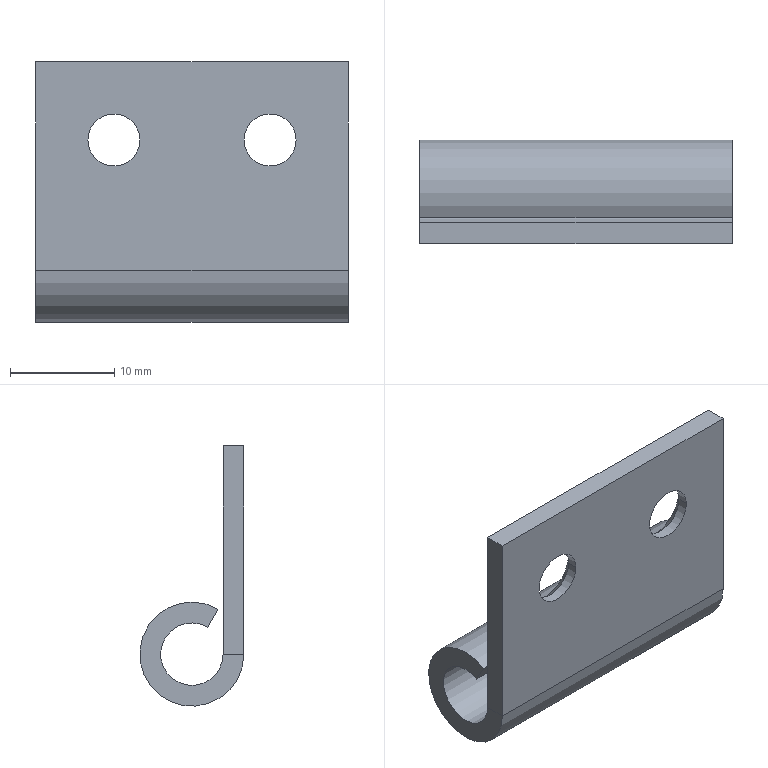Component | SolidWorks | Hinge-1_Hinge2-2 | 1 solid | 18 faces | box 30 x 10 x 25 mm | volume 2360 mm3 | plane 8 | cylinder 6 | cone 4 | commonest cylinder face diameters 5 x4 6 x1 10 x1
STEP:
#1=CARTESIAN_POINT('',(47.055,58.634,58.423));
#2=VERTEX_POINT('',#1);
#3=CARTESIAN_POINT('',(47.251,58.634,58.423));
#4=VERTEX_POINT('',#3);
#5=CARTESIAN_POINT('',(47.153,58.634,58.423));
#6=DIRECTION('',(0.,1.,0.));
#7=DIRECTION('',(1.,0.,0.));
#8=AXIS2_PLACEMENT_3D('',#5,#6,#7);
#9=CIRCLE('',#8,0.09843);
#10=EDGE_CURVE('',#2,#4,#9,.T.);
#11=ORIENTED_EDGE('',*,*,#10,.F.);
#12=CARTESIAN_POINT('',(47.015,58.674,58.423));
#13=VERTEX_POINT('',#12);
#14=CARTESIAN_POINT('',(47.015,58.674,58.423));
#15=DIRECTION('',(-0.7071,0.7071,0.));
#16=VECTOR('',#15,39.37);
#17=LINE('',#14,#16);
#18=EDGE_CURVE('',#2,#13,#17,.T.);
#19=ORIENTED_EDGE('',*,*,#18,.T.);
#20=CARTESIAN_POINT('',(47.291,58.674,58.423));
#21=VERTEX_POINT('',#20);
#22=CARTESIAN_POINT('',(47.153,58.674,58.423));
#23=DIRECTION('',(-0.,-1.,-0.));
#24=DIRECTION('',(1.,0.,0.));
#25=AXIS2_PLACEMENT_3D('',#22,#23,#24);
#26=CIRCLE('',#25,0.1378);
#27=EDGE_CURVE('',#21,#13,#26,.T.);
#28=ORIENTED_EDGE('',*,*,#27,.F.);
#29=CARTESIAN_POINT('',(47.291,58.674,58.423));
#30=DIRECTION('',(0.7071,0.7071,0.));
#31=VECTOR('',#30,39.37);
#32=LINE('',#29,#31);
#33=EDGE_CURVE('',#4,#21,#32,.T.);
#34=ORIENTED_EDGE('',*,*,#33,.F.);
#35=EDGE_LOOP('',(#11,#19,#28,#34));
#36=FACE_OUTER_BOUND('',#35,.T.);
#37=CARTESIAN_POINT('',(47.153,58.674,58.423));
#38=DIRECTION('',(0.,1.,0.));
#39=DIRECTION('',(1.,0.,0.));
#40=AXIS2_PLACEMENT_3D('',#37,#38,#39);
#41=CONICAL_SURFACE('',#40,0.1378,0.7854);
#42=ADVANCED_FACE('',(#36),#41,.F.);
#43=CARTESIAN_POINT('',(46.464,58.634,58.423));
#44=VERTEX_POINT('',#43);
#45=CARTESIAN_POINT('',(46.661,58.634,58.423));
#46=VERTEX_POINT('',#45);
#47=CARTESIAN_POINT('',(46.562,58.634,58.423));
#48=DIRECTION('',(0.,1.,0.));
#49=DIRECTION('',(1.,0.,0.));
#50=AXIS2_PLACEMENT_3D('',#47,#48,#49);
#51=CIRCLE('',#50,0.09843);
#52=EDGE_CURVE('',#44,#46,#51,.T.);
#53=ORIENTED_EDGE('',*,*,#52,.F.);
#54=CARTESIAN_POINT('',(46.425,58.674,58.423));
#55=VERTEX_POINT('',#54);
#56=CARTESIAN_POINT('',(46.425,58.674,58.423));
#57=DIRECTION('',(-0.7071,0.7071,0.));
#58=VECTOR('',#57,39.37);
#59=LINE('',#56,#58);
#60=EDGE_CURVE('',#44,#55,#59,.T.);
#61=ORIENTED_EDGE('',*,*,#60,.T.);
#62=CARTESIAN_POINT('',(46.7,58.674,58.423));
#63=VERTEX_POINT('',#62);
#64=CARTESIAN_POINT('',(46.562,58.674,58.423));
#65=DIRECTION('',(-0.,-1.,-0.));
#66=DIRECTION('',(1.,0.,0.));
#67=AXIS2_PLACEMENT_3D('',#64,#65,#66);
#68=CIRCLE('',#67,0.1378);
#69=EDGE_CURVE('',#63,#55,#68,.T.);
#70=ORIENTED_EDGE('',*,*,#69,.F.);
#71=CARTESIAN_POINT('',(46.7,58.674,58.423));
#72=DIRECTION('',(0.7071,0.7071,0.));
#73=VECTOR('',#72,39.37);
#74=LINE('',#71,#73);
#75=EDGE_CURVE('',#46,#63,#74,.T.);
#76=ORIENTED_EDGE('',*,*,#75,.F.);
#77=EDGE_LOOP('',(#53,#61,#70,#76));
#78=FACE_OUTER_BOUND('',#77,.T.);
#79=CARTESIAN_POINT('',(46.562,58.674,58.423));
#80=DIRECTION('',(0.,1.,0.));
#81=DIRECTION('',(1.,0.,0.));
#82=AXIS2_PLACEMENT_3D('',#79,#80,#81);
#83=CONICAL_SURFACE('',#82,0.1378,0.7854);
#84=ADVANCED_FACE('',(#78),#83,.F.);
#85=ORIENTED_EDGE('',*,*,#10,.T.);
#86=CARTESIAN_POINT('',(47.251,58.595,58.423));
#87=VERTEX_POINT('',#86);
#88=CARTESIAN_POINT('',(47.251,58.989,58.423));
#89=DIRECTION('',(-0.,-1.,-0.));
#90=VECTOR('',#89,39.37);
#91=LINE('',#88,#90);
#92=EDGE_CURVE('',#4,#87,#91,.T.);
#93=ORIENTED_EDGE('',*,*,#92,.T.);
#94=CARTESIAN_POINT('',(47.055,58.595,58.423));
#95=VERTEX_POINT('',#94);
#96=CARTESIAN_POINT('',(47.153,58.595,58.423));
#97=DIRECTION('',(-0.,-1.,-0.));
#98=DIRECTION('',(-1.,0.,0.));
#99=AXIS2_PLACEMENT_3D('',#96,#97,#98);
#100=CIRCLE('',#99,0.09843);
#101=EDGE_CURVE('',#87,#95,#100,.T.);
#102=ORIENTED_EDGE('',*,*,#101,.T.);
#103=CARTESIAN_POINT('',(47.055,58.989,58.423));
#104=DIRECTION('',(-0.,-1.,-0.));
#105=VECTOR('',#104,39.37);
#106=LINE('',#103,#105);
#107=EDGE_CURVE('',#2,#95,#106,.T.);
#108=ORIENTED_EDGE('',*,*,#107,.F.);
#109=EDGE_LOOP('',(#85,#93,#102,#108));
#110=FACE_OUTER_BOUND('',#109,.T.);
#111=CARTESIAN_POINT('',(47.153,58.989,58.423));
#112=DIRECTION('',(-0.,-1.,-0.));
#113=DIRECTION('',(-1.,0.,0.));
#114=AXIS2_PLACEMENT_3D('',#111,#112,#113);
#115=CYLINDRICAL_SURFACE('',#114,0.09843);
#116=ADVANCED_FACE('',(#110),#115,.F.);
#117=ORIENTED_EDGE('',*,*,#52,.T.);
#118=CARTESIAN_POINT('',(46.661,58.595,58.423));
#119=VERTEX_POINT('',#118);
#120=CARTESIAN_POINT('',(46.661,58.989,58.423));
#121=DIRECTION('',(-0.,-1.,-0.));
#122=VECTOR('',#121,39.37);
#123=LINE('',#120,#122);
#124=EDGE_CURVE('',#46,#119,#123,.T.);
#125=ORIENTED_EDGE('',*,*,#124,.T.);
#126=CARTESIAN_POINT('',(46.464,58.595,58.423));
#127=VERTEX_POINT('',#126);
#128=CARTESIAN_POINT('',(46.562,58.595,58.423));
#129=DIRECTION('',(-0.,-1.,-0.));
#130=DIRECTION('',(-1.,0.,0.));
#131=AXIS2_PLACEMENT_3D('',#128,#129,#130);
#132=CIRCLE('',#131,0.09843);
#133=EDGE_CURVE('',#119,#127,#132,.T.);
#134=ORIENTED_EDGE('',*,*,#133,.T.);
#135=CARTESIAN_POINT('',(46.464,58.989,58.423));
#136=DIRECTION('',(-0.,-1.,-0.));
#137=VECTOR('',#136,39.37);
#138=LINE('',#135,#137);
#139=EDGE_CURVE('',#44,#127,#138,.T.);
#140=ORIENTED_EDGE('',*,*,#139,.F.);
#141=EDGE_LOOP('',(#117,#125,#134,#140));
#142=FACE_OUTER_BOUND('',#141,.T.);
#143=CARTESIAN_POINT('',(46.562,58.989,58.423));
#144=DIRECTION('',(-0.,-1.,-0.));
#145=DIRECTION('',(-1.,0.,0.));
#146=AXIS2_PLACEMENT_3D('',#143,#144,#145);
#147=CYLINDRICAL_SURFACE('',#146,0.09843);
#148=ADVANCED_FACE('',(#142),#147,.F.);
#149=CARTESIAN_POINT('',(46.267,58.674,57.931));
#150=VERTEX_POINT('',#149);
#151=CARTESIAN_POINT('',(46.267,58.595,57.931));
#152=VERTEX_POINT('',#151);
#153=CARTESIAN_POINT('',(46.267,58.674,57.931));
#154=DIRECTION('',(-0.,-1.,-0.));
#155=VECTOR('',#154,39.37);
#156=LINE('',#153,#155);
#157=EDGE_CURVE('',#150,#152,#156,.T.);
#158=ORIENTED_EDGE('',*,*,#157,.F.);
#159=CARTESIAN_POINT('',(46.267,58.733,58.034));
#160=VERTEX_POINT('',#159);
#161=CARTESIAN_POINT('',(46.267,58.792,57.931));
#162=DIRECTION('',(-1.,0.,0.));
#163=DIRECTION('',(0.,1.,0.));
#164=AXIS2_PLACEMENT_3D('',#161,#162,#163);
#165=CIRCLE('',#164,0.1181);
#166=EDGE_CURVE('',#160,#150,#165,.T.);
#167=ORIENTED_EDGE('',*,*,#166,.F.);
#168=CARTESIAN_POINT('',(46.267,58.693,58.102));
#169=VERTEX_POINT('',#168);
#170=CARTESIAN_POINT('',(46.267,58.693,58.102));
#171=DIRECTION('',(0.,0.5,-0.866));
#172=VECTOR('',#171,39.37);
#173=LINE('',#170,#172);
#174=EDGE_CURVE('',#169,#160,#173,.T.);
#175=ORIENTED_EDGE('',*,*,#174,.F.);
#176=CARTESIAN_POINT('',(46.267,58.792,57.931));
#177=DIRECTION('',(-1.,0.,0.));
#178=DIRECTION('',(0.,1.,0.));
#179=AXIS2_PLACEMENT_3D('',#176,#177,#178);
#180=CIRCLE('',#179,0.1969);
#181=EDGE_CURVE('',#169,#152,#180,.T.);
#182=ORIENTED_EDGE('',*,*,#181,.T.);
#183=EDGE_LOOP('',(#158,#167,#175,#182));
#184=FACE_OUTER_BOUND('',#183,.T.);
#185=CARTESIAN_POINT('',(46.267,58.674,57.931));
#186=DIRECTION('',(-1.,0.,0.));
#187=DIRECTION('',(0.,1.,0.));
#188=AXIS2_PLACEMENT_3D('',#185,#186,#187);
#189=PLANE('',#188);
#190=ADVANCED_FACE('',(#184),#189,.T.);
#191=CARTESIAN_POINT('',(47.448,58.595,57.931));
#192=VERTEX_POINT('',#191);
#193=CARTESIAN_POINT('',(47.448,58.674,57.931));
#194=VERTEX_POINT('',#193);
#195=CARTESIAN_POINT('',(47.448,58.595,57.931));
#196=DIRECTION('',(0.,1.,0.));
#197=VECTOR('',#196,39.37);
#198=LINE('',#195,#197);
#199=EDGE_CURVE('',#192,#194,#198,.T.);
#200=ORIENTED_EDGE('',*,*,#199,.F.);
#201=CARTESIAN_POINT('',(47.448,58.693,58.102));
#202=VERTEX_POINT('',#201);
#203=CARTESIAN_POINT('',(47.448,58.792,57.931));
#204=DIRECTION('',(-1.,0.,0.));
#205=DIRECTION('',(0.,1.,0.));
#206=AXIS2_PLACEMENT_3D('',#203,#204,#205);
#207=CIRCLE('',#206,0.1969);
#208=EDGE_CURVE('',#202,#192,#207,.T.);
#209=ORIENTED_EDGE('',*,*,#208,.F.);
#210=CARTESIAN_POINT('',(47.448,58.733,58.034));
#211=VERTEX_POINT('',#210);
#212=CARTESIAN_POINT('',(47.448,58.693,58.102));
#213=DIRECTION('',(0.,0.5,-0.866));
#214=VECTOR('',#213,39.37);
#215=LINE('',#212,#214);
#216=EDGE_CURVE('',#202,#211,#215,.T.);
#217=ORIENTED_EDGE('',*,*,#216,.T.);
#218=CARTESIAN_POINT('',(47.448,58.792,57.931));
#219=DIRECTION('',(-1.,0.,0.));
#220=DIRECTION('',(0.,1.,0.));
#221=AXIS2_PLACEMENT_3D('',#218,#219,#220);
#222=CIRCLE('',#221,0.1181);
#223=EDGE_CURVE('',#211,#194,#222,.T.);
#224=ORIENTED_EDGE('',*,*,#223,.T.);
#225=EDGE_LOOP('',(#200,#209,#217,#224));
#226=FACE_OUTER_BOUND('',#225,.T.);
#227=CARTESIAN_POINT('',(47.448,58.595,57.931));
#228=DIRECTION('',(1.,-0.,-0.));
#229=DIRECTION('',(-0.,-1.,-0.));
#230=AXIS2_PLACEMENT_3D('',#227,#228,#229);
#231=PLANE('',#230);
#232=ADVANCED_FACE('',(#226),#231,.T.);
#233=CARTESIAN_POINT('',(47.153,58.595,58.423));
#234=DIRECTION('',(-0.,-1.,-0.));
#235=DIRECTION('',(-1.,0.,0.));
#236=AXIS2_PLACEMENT_3D('',#233,#234,#235);
#237=CIRCLE('',#236,0.09843);
#238=EDGE_CURVE('',#95,#87,#237,.T.);
#239=ORIENTED_EDGE('',*,*,#238,.F.);
#240=ORIENTED_EDGE('',*,*,#101,.F.);
#241=EDGE_LOOP('',(#239,#240));
#242=FACE_BOUND('',#241,.T.);
#243=CARTESIAN_POINT('',(46.562,58.595,58.423));
#244=DIRECTION('',(-0.,-1.,-0.));
#245=DIRECTION('',(-1.,0.,0.));
#246=AXIS2_PLACEMENT_3D('',#243,#244,#245);
#247=CIRCLE('',#246,0.09843);
#248=EDGE_CURVE('',#127,#119,#247,.T.);
#249=ORIENTED_EDGE('',*,*,#248,.F.);
#250=ORIENTED_EDGE('',*,*,#133,.F.);
#251=EDGE_LOOP('',(#249,#250));
#252=FACE_BOUND('',#251,.T.);
#253=CARTESIAN_POINT('',(47.448,58.595,58.719));
#254=VERTEX_POINT('',#253);
#255=CARTESIAN_POINT('',(47.448,58.595,58.719));
#256=DIRECTION('',(0.,-0.,1.));
#257=VECTOR('',#256,39.37);
#258=LINE('',#255,#257);
#259=EDGE_CURVE('',#192,#254,#258,.T.);
#260=ORIENTED_EDGE('',*,*,#259,.T.);
#261=CARTESIAN_POINT('',(46.267,58.595,58.719));
#262=VERTEX_POINT('',#261);
#263=CARTESIAN_POINT('',(46.267,58.595,58.719));
#264=DIRECTION('',(1.,-0.,-0.));
#265=VECTOR('',#264,39.37);
#266=LINE('',#263,#265);
#267=EDGE_CURVE('',#262,#254,#266,.T.);
#268=ORIENTED_EDGE('',*,*,#267,.F.);
#269=CARTESIAN_POINT('',(46.267,58.595,58.719));
#270=DIRECTION('',(0.,-0.,1.));
#271=VECTOR('',#270,39.37);
#272=LINE('',#269,#271);
#273=EDGE_CURVE('',#152,#262,#272,.T.);
#274=ORIENTED_EDGE('',*,*,#273,.F.);
#275=CARTESIAN_POINT('',(46.267,58.595,57.931));
#276=DIRECTION('',(1.,-0.,-0.));
#277=VECTOR('',#276,39.37);
#278=LINE('',#275,#277);
#279=EDGE_CURVE('',#152,#192,#278,.T.);
#280=ORIENTED_EDGE('',*,*,#279,.T.);
#281=EDGE_LOOP('',(#260,#268,#274,#280));
#282=FACE_OUTER_BOUND('',#281,.T.);
#283=CARTESIAN_POINT('',(46.267,58.595,58.719));
#284=DIRECTION('',(0.,1.,0.));
#285=DIRECTION('',(1.,-0.,-0.));
#286=AXIS2_PLACEMENT_3D('',#283,#284,#285);
#287=PLANE('',#286);
#288=ADVANCED_FACE('',(#242,#252,#282),#287,.F.);
#289=CARTESIAN_POINT('',(47.448,58.674,58.719));
#290=VERTEX_POINT('',#289);
#291=CARTESIAN_POINT('',(47.448,58.674,58.719));
#292=DIRECTION('',(-0.,-1.,-0.));
#293=VECTOR('',#292,39.37);
#294=LINE('',#291,#293);
#295=EDGE_CURVE('',#290,#254,#294,.T.);
#296=ORIENTED_EDGE('',*,*,#295,.F.);
#297=CARTESIAN_POINT('',(46.267,58.674,58.719));
#298=VERTEX_POINT('',#297);
#299=CARTESIAN_POINT('',(46.267,58.674,58.719));
#300=DIRECTION('',(1.,-0.,-0.));
#301=VECTOR('',#300,39.37);
#302=LINE('',#299,#301);
#303=EDGE_CURVE('',#298,#290,#302,.T.);
#304=ORIENTED_EDGE('',*,*,#303,.F.);
#305=CARTESIAN_POINT('',(46.267,58.674,58.719));
#306=DIRECTION('',(-0.,-1.,-0.));
#307=VECTOR('',#306,39.37);
#308=LINE('',#305,#307);
#309=EDGE_CURVE('',#298,#262,#308,.T.);
#310=ORIENTED_EDGE('',*,*,#309,.T.);
#311=ORIENTED_EDGE('',*,*,#267,.T.);
#312=EDGE_LOOP('',(#296,#304,#310,#311));
#313=FACE_OUTER_BOUND('',#312,.T.);
#314=CARTESIAN_POINT('',(46.267,58.674,58.719));
#315=DIRECTION('',(0.,-0.,1.));
#316=DIRECTION('',(0.,1.,0.));
#317=AXIS2_PLACEMENT_3D('',#314,#315,#316);
#318=PLANE('',#317);
#319=ADVANCED_FACE('',(#313),#318,.T.);
#320=ORIENTED_EDGE('',*,*,#69,.T.);
#321=CARTESIAN_POINT('',(46.562,58.674,58.423));
#322=DIRECTION('',(-0.,-1.,-0.));
#323=DIRECTION('',(1.,0.,0.));
#324=AXIS2_PLACEMENT_3D('',#321,#322,#323);
#325=CIRCLE('',#324,0.1378);
#326=EDGE_CURVE('',#55,#63,#325,.T.);
#327=ORIENTED_EDGE('',*,*,#326,.T.);
#328=EDGE_LOOP('',(#320,#327));
#329=FACE_BOUND('',#328,.T.);
#330=ORIENTED_EDGE('',*,*,#27,.T.);
#331=CARTESIAN_POINT('',(47.153,58.674,58.423));
#332=DIRECTION('',(-0.,-1.,-0.));
#333=DIRECTION('',(1.,0.,0.));
#334=AXIS2_PLACEMENT_3D('',#331,#332,#333);
#335=CIRCLE('',#334,0.1378);
#336=EDGE_CURVE('',#13,#21,#335,.T.);
#337=ORIENTED_EDGE('',*,*,#336,.T.);
#338=EDGE_LOOP('',(#330,#337));
#339=FACE_BOUND('',#338,.T.);
#340=CARTESIAN_POINT('',(47.448,58.674,58.719));
#341=DIRECTION('',(0.,-0.,1.));
#342=VECTOR('',#341,39.37);
#343=LINE('',#340,#342);
#344=EDGE_CURVE('',#194,#290,#343,.T.);
#345=ORIENTED_EDGE('',*,*,#344,.F.);
#346=CARTESIAN_POINT('',(46.267,58.674,57.931));
#347=DIRECTION('',(1.,-0.,-0.));
#348=VECTOR('',#347,39.37);
#349=LINE('',#346,#348);
#350=EDGE_CURVE('',#150,#194,#349,.T.);
#351=ORIENTED_EDGE('',*,*,#350,.F.);
#352=CARTESIAN_POINT('',(46.267,58.674,58.719));
#353=DIRECTION('',(0.,-0.,1.));
#354=VECTOR('',#353,39.37);
#355=LINE('',#352,#354);
#356=EDGE_CURVE('',#150,#298,#355,.T.);
#357=ORIENTED_EDGE('',*,*,#356,.T.);
#358=ORIENTED_EDGE('',*,*,#303,.T.);
#359=EDGE_LOOP('',(#345,#351,#357,#358));
#360=FACE_OUTER_BOUND('',#359,.T.);
#361=CARTESIAN_POINT('',(46.267,58.674,58.719));
#362=DIRECTION('',(0.,1.,0.));
#363=DIRECTION('',(1.,-0.,-0.));
#364=AXIS2_PLACEMENT_3D('',#361,#362,#363);
#365=PLANE('',#364);
#366=ADVANCED_FACE('',(#329,#339,#360),#365,.T.);
#367=ORIENTED_EDGE('',*,*,#223,.F.);
#368=CARTESIAN_POINT('',(46.267,58.733,58.034));
#369=DIRECTION('',(1.,-0.,-0.));
#370=VECTOR('',#369,39.37);
#371=LINE('',#368,#370);
#372=EDGE_CURVE('',#160,#211,#371,.T.);
#373=ORIENTED_EDGE('',*,*,#372,.F.);
#374=ORIENTED_EDGE('',*,*,#166,.T.);
#375=ORIENTED_EDGE('',*,*,#350,.T.);
#376=EDGE_LOOP('',(#367,#373,#374,#375));
#377=FACE_OUTER_BOUND('',#376,.T.);
#378=CARTESIAN_POINT('',(46.267,58.792,57.931));
#379=DIRECTION('',(1.,-0.,-0.));
#380=DIRECTION('',(0.,-1.,0.));
#381=AXIS2_PLACEMENT_3D('',#378,#379,#380);
#382=CYLINDRICAL_SURFACE('',#381,0.1181);
#383=ADVANCED_FACE('',(#377),#382,.F.);
#384=ORIENTED_EDGE('',*,*,#216,.F.);
#385=CARTESIAN_POINT('',(46.267,58.693,58.102));
#386=DIRECTION('',(1.,-0.,-0.));
#387=VECTOR('',#386,39.37);
#388=LINE('',#385,#387);
#389=EDGE_CURVE('',#169,#202,#388,.T.);
#390=ORIENTED_EDGE('',*,*,#389,.F.);
#391=ORIENTED_EDGE('',*,*,#174,.T.);
#392=ORIENTED_EDGE('',*,*,#372,.T.);
#393=EDGE_LOOP('',(#384,#390,#391,#392));
#394=FACE_OUTER_BOUND('',#393,.T.);
#395=CARTESIAN_POINT('',(46.267,58.693,58.102));
#396=DIRECTION('',(-0.,-0.866,-0.5));
#397=DIRECTION('',(-0.,-0.5,0.866));
#398=AXIS2_PLACEMENT_3D('',#395,#396,#397);
#399=PLANE('',#398);
#400=ADVANCED_FACE('',(#394),#399,.T.);
#401=ORIENTED_EDGE('',*,*,#208,.T.);
#402=ORIENTED_EDGE('',*,*,#279,.F.);
#403=ORIENTED_EDGE('',*,*,#181,.F.);
#404=ORIENTED_EDGE('',*,*,#389,.T.);
#405=EDGE_LOOP('',(#401,#402,#403,#404));
#406=FACE_OUTER_BOUND('',#405,.T.);
#407=CARTESIAN_POINT('',(46.267,58.792,57.931));
#408=DIRECTION('',(1.,-0.,-0.));
#409=DIRECTION('',(0.,-1.,0.));
#410=AXIS2_PLACEMENT_3D('',#407,#408,#409);
#411=CYLINDRICAL_SURFACE('',#410,0.1969);
#412=ADVANCED_FACE('',(#406),#411,.T.);
#413=ORIENTED_EDGE('',*,*,#273,.T.);
#414=ORIENTED_EDGE('',*,*,#309,.F.);
#415=ORIENTED_EDGE('',*,*,#356,.F.);
#416=ORIENTED_EDGE('',*,*,#157,.T.);
#417=EDGE_LOOP('',(#413,#414,#415,#416));
#418=FACE_OUTER_BOUND('',#417,.T.);
#419=CARTESIAN_POINT('',(46.267,58.792,57.931));
#420=DIRECTION('',(-1.,0.,0.));
#421=DIRECTION('',(0.,1.,0.));
#422=AXIS2_PLACEMENT_3D('',#419,#420,#421);
#423=PLANE('',#422);
#424=ADVANCED_FACE('',(#418),#423,.T.);
#425=ORIENTED_EDGE('',*,*,#259,.F.);
#426=ORIENTED_EDGE('',*,*,#199,.T.);
#427=ORIENTED_EDGE('',*,*,#344,.T.);
#428=ORIENTED_EDGE('',*,*,#295,.T.);
#429=EDGE_LOOP('',(#425,#426,#427,#428));
#430=FACE_OUTER_BOUND('',#429,.T.);
#431=CARTESIAN_POINT('',(47.448,58.792,57.931));
#432=DIRECTION('',(-1.,0.,0.));
#433=DIRECTION('',(0.,1.,0.));
#434=AXIS2_PLACEMENT_3D('',#431,#432,#433);
#435=PLANE('',#434);
#436=ADVANCED_FACE('',(#430),#435,.F.);
#437=ORIENTED_EDGE('',*,*,#124,.F.);
#438=CARTESIAN_POINT('',(46.562,58.634,58.423));
#439=DIRECTION('',(0.,1.,0.));
#440=DIRECTION('',(1.,0.,0.));
#441=AXIS2_PLACEMENT_3D('',#438,#439,#440);
#442=CIRCLE('',#441,0.09843);
#443=EDGE_CURVE('',#46,#44,#442,.T.);
#444=ORIENTED_EDGE('',*,*,#443,.T.);
#445=ORIENTED_EDGE('',*,*,#139,.T.);
#446=ORIENTED_EDGE('',*,*,#248,.T.);
#447=EDGE_LOOP('',(#437,#444,#445,#446));
#448=FACE_OUTER_BOUND('',#447,.T.);
#449=CARTESIAN_POINT('',(46.562,58.989,58.423));
#450=DIRECTION('',(-0.,-1.,-0.));
#451=DIRECTION('',(-1.,0.,0.));
#452=AXIS2_PLACEMENT_3D('',#449,#450,#451);
#453=CYLINDRICAL_SURFACE('',#452,0.09843);
#454=ADVANCED_FACE('',(#448),#453,.F.);
#455=ORIENTED_EDGE('',*,*,#92,.F.);
#456=CARTESIAN_POINT('',(47.153,58.634,58.423));
#457=DIRECTION('',(0.,1.,0.));
#458=DIRECTION('',(1.,0.,0.));
#459=AXIS2_PLACEMENT_3D('',#456,#457,#458);
#460=CIRCLE('',#459,0.09843);
#461=EDGE_CURVE('',#4,#2,#460,.T.);
#462=ORIENTED_EDGE('',*,*,#461,.T.);
#463=ORIENTED_EDGE('',*,*,#107,.T.);
#464=ORIENTED_EDGE('',*,*,#238,.T.);
#465=EDGE_LOOP('',(#455,#462,#463,#464));
#466=FACE_OUTER_BOUND('',#465,.T.);
#467=CARTESIAN_POINT('',(47.153,58.989,58.423));
#468=DIRECTION('',(-0.,-1.,-0.));
#469=DIRECTION('',(-1.,0.,0.));
#470=AXIS2_PLACEMENT_3D('',#467,#468,#469);
#471=CYLINDRICAL_SURFACE('',#470,0.09843);
#472=ADVANCED_FACE('',(#466),#471,.F.);
#473=ORIENTED_EDGE('',*,*,#60,.F.);
#474=ORIENTED_EDGE('',*,*,#443,.F.);
#475=ORIENTED_EDGE('',*,*,#75,.T.);
#476=ORIENTED_EDGE('',*,*,#326,.F.);
#477=EDGE_LOOP('',(#473,#474,#475,#476));
#478=FACE_OUTER_BOUND('',#477,.T.);
#479=CARTESIAN_POINT('',(46.562,58.674,58.423));
#480=DIRECTION('',(0.,1.,0.));
#481=DIRECTION('',(1.,0.,0.));
#482=AXIS2_PLACEMENT_3D('',#479,#480,#481);
#483=CONICAL_SURFACE('',#482,0.1378,0.7854);
#484=ADVANCED_FACE('',(#478),#483,.F.);
#485=ORIENTED_EDGE('',*,*,#18,.F.);
#486=ORIENTED_EDGE('',*,*,#461,.F.);
#487=ORIENTED_EDGE('',*,*,#33,.T.);
#488=ORIENTED_EDGE('',*,*,#336,.F.);
#489=EDGE_LOOP('',(#485,#486,#487,#488));
#490=FACE_OUTER_BOUND('',#489,.T.);
#491=CARTESIAN_POINT('',(47.153,58.674,58.423));
#492=DIRECTION('',(0.,1.,0.));
#493=DIRECTION('',(1.,0.,0.));
#494=AXIS2_PLACEMENT_3D('',#491,#492,#493);
#495=CONICAL_SURFACE('',#494,0.1378,0.7854);
#496=ADVANCED_FACE('',(#490),#495,.F.);
#497=CLOSED_SHELL('',(#42,#84,#116,#148,#190,#232,#288,#319,#366,#383,#400,#412,#424,#436,#454,#472,#484,#496));
#498=MANIFOLD_SOLID_BREP('',#497);
#499=CARTESIAN_POINT('',(0.,0.,0.));
#500=DIRECTION('',(0.,0.,1.));
#501=DIRECTION('',(1.,0.,0.));
#502=AXIS2_PLACEMENT_3D('',#499,#500,#501);
#503=(LENGTH_UNIT()NAMED_UNIT(*)SI_UNIT($,.METRE.));
#504=LENGTH_MEASURE_WITH_UNIT(LENGTH_MEASURE(0.0254),#503);
#505=DIMENSIONAL_EXPONENTS(1.,0.,0.,0.,0.,0.,0.);
#506=(CONVERSION_BASED_UNIT('',#504)LENGTH_UNIT()NAMED_UNIT(#505));
#507=UNCERTAINTY_MEASURE_WITH_UNIT(LENGTH_MEASURE(0.00001),#506,'','');
#508=(NAMED_UNIT(*)PLANE_ANGLE_UNIT()SI_UNIT($,.RADIAN.));
#509=(NAMED_UNIT(*)SI_UNIT($,.STERADIAN.)SOLID_ANGLE_UNIT());
#510=(GEOMETRIC_REPRESENTATION_CONTEXT(3)GLOBAL_UNCERTAINTY_ASSIGNED_CONTEXT((#507))GLOBAL_UNIT_ASSIGNED_CONTEXT((#506,#508,#509))REPRESENTATION_CONTEXT('',''));
#511=ADVANCED_BREP_SHAPE_REPRESENTATION('',(#498,#502),#510);
#512=COLOUR_RGB('',0.7922,0.8196,0.9333);
#513=FILL_AREA_STYLE_COLOUR('',#512);
#514=FILL_AREA_STYLE('',(#513));
#515=SURFACE_STYLE_FILL_AREA(#514);
#516=SURFACE_SIDE_STYLE('',(#515));
#517=SURFACE_STYLE_USAGE(.BOTH.,#516);
#518=PRESENTATION_STYLE_ASSIGNMENT((#517));
#519=STYLED_ITEM('',(#518),#498);
#520=(LENGTH_UNIT()NAMED_UNIT(*)SI_UNIT($,.METRE.));
#521=LENGTH_MEASURE_WITH_UNIT(LENGTH_MEASURE(0.0254),#520);
#522=DIMENSIONAL_EXPONENTS(1.,0.,0.,0.,0.,0.,0.);
#523=(CONVERSION_BASED_UNIT('',#521)LENGTH_UNIT()NAMED_UNIT(#522));
#524=UNCERTAINTY_MEASURE_WITH_UNIT(LENGTH_MEASURE(0.00001),#523,'','');
#525=(NAMED_UNIT(*)PLANE_ANGLE_UNIT()SI_UNIT($,.RADIAN.));
#526=(NAMED_UNIT(*)SI_UNIT($,.STERADIAN.)SOLID_ANGLE_UNIT());
#527=(GEOMETRIC_REPRESENTATION_CONTEXT(3)GLOBAL_UNCERTAINTY_ASSIGNED_CONTEXT((#524))GLOBAL_UNIT_ASSIGNED_CONTEXT((#523,#525,#526))REPRESENTATION_CONTEXT('',''));
#528=MECHANICAL_DESIGN_GEOMETRIC_PRESENTATION_REPRESENTATION('',(#519),#527);
#529=PRESENTATION_LAYER_ASSIGNMENT('','',(#519));